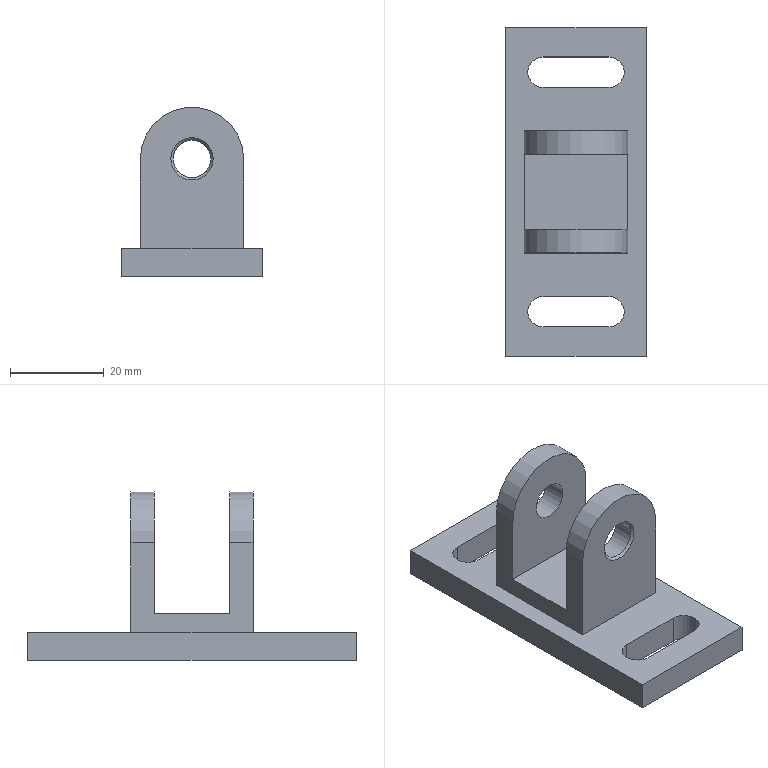Component | NX | FIXED_MOUNT | 1 solid | 26 faces | volume 18093 mm3 | plane 17 | cylinder 8 | cone 1 | commonest cylinder face diameters 6.5 x4 22 x2 8 x2